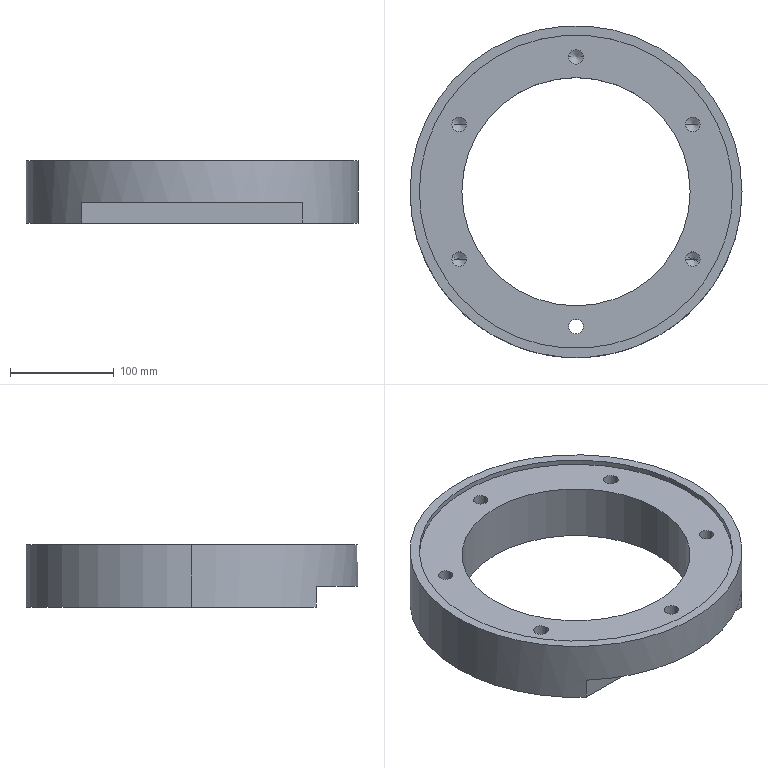Component | SolidWorks | JF21-80.1-1-3(_)-1-SOLID31-1 | 1 solid | 33 faces | box 320 x 320 x 60 mm | volume 2225570 mm3 | cylinder 18 | cone 10 | plane 5 | commonest cylinder face diameters 14 x12 302 x2 320 x2 220 x2
STEP:
#1=COLOUR_RGB('',0.7922,0.8196,0.9333);
#2=FILL_AREA_STYLE_COLOUR('',#1);
#3=FILL_AREA_STYLE('',(#2));
#4=SURFACE_STYLE_FILL_AREA(#3);
#5=SURFACE_SIDE_STYLE('',(#4));
#6=SURFACE_STYLE_USAGE(.BOTH.,#5);
#7=PRESENTATION_STYLE_ASSIGNMENT((#6));
#8=CARTESIAN_POINT('',(-4.708,-13.039,24.961));
#9=VERTEX_POINT('',#8);
#10=CARTESIAN_POINT('',(-4.157,-13.039,24.961));
#11=VERTEX_POINT('',#10);
#12=CARTESIAN_POINT('',(-4.432,-13.039,24.961));
#13=DIRECTION('',(0.,0.,1.));
#14=DIRECTION('',(1.,0.,0.));
#15=AXIS2_PLACEMENT_3D('',#12,#13,#14);
#16=CIRCLE('',#15,0.2756);
#17=EDGE_CURVE('',#9,#11,#16,.T.);
#18=ORIENTED_EDGE('',*,*,#17,.F.);
#19=CARTESIAN_POINT('',(-4.708,-13.039,26.378));
#20=VERTEX_POINT('',#19);
#21=CARTESIAN_POINT('',(-4.708,-13.039,26.378));
#22=DIRECTION('',(0.,0.,1.));
#23=VECTOR('',#22,39.37);
#24=LINE('',#21,#23);
#25=EDGE_CURVE('',#9,#20,#24,.T.);
#26=ORIENTED_EDGE('',*,*,#25,.T.);
#27=CARTESIAN_POINT('',(-4.157,-13.039,26.378));
#28=VERTEX_POINT('',#27);
#29=CARTESIAN_POINT('',(-4.432,-13.039,26.378));
#30=DIRECTION('',(0.,0.,1.));
#31=DIRECTION('',(1.,0.,0.));
#32=AXIS2_PLACEMENT_3D('',#29,#30,#31);
#33=CIRCLE('',#32,0.2756);
#34=EDGE_CURVE('',#20,#28,#33,.T.);
#35=ORIENTED_EDGE('',*,*,#34,.T.);
#36=CARTESIAN_POINT('',(-4.157,-13.039,26.378));
#37=DIRECTION('',(0.,0.,1.));
#38=VECTOR('',#37,39.37);
#39=LINE('',#36,#38);
#40=EDGE_CURVE('',#11,#28,#39,.T.);
#41=ORIENTED_EDGE('',*,*,#40,.F.);
#42=EDGE_LOOP('',(#18,#26,#35,#41));
#43=FACE_OUTER_BOUND('',#42,.T.);
#44=CARTESIAN_POINT('',(-4.432,-13.039,26.378));
#45=DIRECTION('',(0.,0.,1.));
#46=DIRECTION('',(-1.,0.,0.));
#47=AXIS2_PLACEMENT_3D('',#44,#45,#46);
#48=CYLINDRICAL_SURFACE('',#47,0.2756);
#49=ADVANCED_FACE('',(#43),#48,.F.);
#50=CARTESIAN_POINT('',(-4.432,-13.039,24.795));
#51=VERTEX_POINT('',#50);
#52=CARTESIAN_POINT('',(-4.157,-13.039,24.961));
#53=DIRECTION('',(0.8572,0.,0.515));
#54=VECTOR('',#53,39.37);
#55=LINE('',#52,#54);
#56=EDGE_CURVE('',#51,#11,#55,.T.);
#57=ORIENTED_EDGE('',*,*,#56,.F.);
#58=CARTESIAN_POINT('',(-4.708,-13.039,24.961));
#59=DIRECTION('',(-0.8572,0.,0.515));
#60=VECTOR('',#59,39.37);
#61=LINE('',#58,#60);
#62=EDGE_CURVE('',#51,#9,#61,.T.);
#63=ORIENTED_EDGE('',*,*,#62,.T.);
#64=ORIENTED_EDGE('',*,*,#17,.T.);
#65=EDGE_LOOP('',(#57,#63,#64));
#66=FACE_OUTER_BOUND('',#65,.T.);
#67=CARTESIAN_POINT('',(-4.432,-13.039,24.961));
#68=DIRECTION('',(0.,0.,1.));
#69=DIRECTION('',(-1.,0.,0.));
#70=AXIS2_PLACEMENT_3D('',#67,#68,#69);
#71=CONICAL_SURFACE('',#70,0.2756,1.03);
#72=ADVANCED_FACE('',(#66),#71,.F.);
#73=CARTESIAN_POINT('',(-4.708,-18.157,24.961));
#74=VERTEX_POINT('',#73);
#75=CARTESIAN_POINT('',(-4.157,-18.157,24.961));
#76=VERTEX_POINT('',#75);
#77=CARTESIAN_POINT('',(-4.432,-18.157,24.961));
#78=DIRECTION('',(0.,0.,1.));
#79=DIRECTION('',(1.,0.,0.));
#80=AXIS2_PLACEMENT_3D('',#77,#78,#79);
#81=CIRCLE('',#80,0.2756);
#82=EDGE_CURVE('',#74,#76,#81,.T.);
#83=ORIENTED_EDGE('',*,*,#82,.F.);
#84=CARTESIAN_POINT('',(-4.708,-18.157,26.378));
#85=VERTEX_POINT('',#84);
#86=CARTESIAN_POINT('',(-4.708,-18.157,26.378));
#87=DIRECTION('',(0.,0.,1.));
#88=VECTOR('',#87,39.37);
#89=LINE('',#86,#88);
#90=EDGE_CURVE('',#74,#85,#89,.T.);
#91=ORIENTED_EDGE('',*,*,#90,.T.);
#92=CARTESIAN_POINT('',(-4.157,-18.157,26.378));
#93=VERTEX_POINT('',#92);
#94=CARTESIAN_POINT('',(-4.432,-18.157,26.378));
#95=DIRECTION('',(0.,0.,1.));
#96=DIRECTION('',(1.,0.,0.));
#97=AXIS2_PLACEMENT_3D('',#94,#95,#96);
#98=CIRCLE('',#97,0.2756);
#99=EDGE_CURVE('',#85,#93,#98,.T.);
#100=ORIENTED_EDGE('',*,*,#99,.T.);
#101=CARTESIAN_POINT('',(-4.157,-18.157,26.378));
#102=DIRECTION('',(0.,0.,1.));
#103=VECTOR('',#102,39.37);
#104=LINE('',#101,#103);
#105=EDGE_CURVE('',#76,#93,#104,.T.);
#106=ORIENTED_EDGE('',*,*,#105,.F.);
#107=EDGE_LOOP('',(#83,#91,#100,#106));
#108=FACE_OUTER_BOUND('',#107,.T.);
#109=CARTESIAN_POINT('',(-4.432,-18.157,26.378));
#110=DIRECTION('',(0.,0.,1.));
#111=DIRECTION('',(-1.,0.,0.));
#112=AXIS2_PLACEMENT_3D('',#109,#110,#111);
#113=CYLINDRICAL_SURFACE('',#112,0.2756);
#114=ADVANCED_FACE('',(#108),#113,.F.);
#115=CARTESIAN_POINT('',(-4.432,-18.157,24.795));
#116=VERTEX_POINT('',#115);
#117=CARTESIAN_POINT('',(-4.157,-18.157,24.961));
#118=DIRECTION('',(0.8572,0.,0.515));
#119=VECTOR('',#118,39.37);
#120=LINE('',#117,#119);
#121=EDGE_CURVE('',#116,#76,#120,.T.);
#122=ORIENTED_EDGE('',*,*,#121,.F.);
#123=CARTESIAN_POINT('',(-4.708,-18.157,24.961));
#124=DIRECTION('',(-0.8572,0.,0.515));
#125=VECTOR('',#124,39.37);
#126=LINE('',#123,#125);
#127=EDGE_CURVE('',#116,#74,#126,.T.);
#128=ORIENTED_EDGE('',*,*,#127,.T.);
#129=ORIENTED_EDGE('',*,*,#82,.T.);
#130=EDGE_LOOP('',(#122,#128,#129));
#131=FACE_OUTER_BOUND('',#130,.T.);
#132=CARTESIAN_POINT('',(-4.432,-18.157,24.961));
#133=DIRECTION('',(0.,0.,1.));
#134=DIRECTION('',(-1.,0.,0.));
#135=AXIS2_PLACEMENT_3D('',#132,#133,#134);
#136=CONICAL_SURFACE('',#135,0.2756,1.03);
#137=ADVANCED_FACE('',(#131),#136,.F.);
#138=CARTESIAN_POINT('',(4.157,-18.157,24.961));
#139=VERTEX_POINT('',#138);
#140=CARTESIAN_POINT('',(4.708,-18.157,24.961));
#141=VERTEX_POINT('',#140);
#142=CARTESIAN_POINT('',(4.432,-18.157,24.961));
#143=DIRECTION('',(0.,0.,1.));
#144=DIRECTION('',(1.,0.,0.));
#145=AXIS2_PLACEMENT_3D('',#142,#143,#144);
#146=CIRCLE('',#145,0.2756);
#147=EDGE_CURVE('',#139,#141,#146,.T.);
#148=ORIENTED_EDGE('',*,*,#147,.F.);
#149=CARTESIAN_POINT('',(4.157,-18.157,26.378));
#150=VERTEX_POINT('',#149);
#151=CARTESIAN_POINT('',(4.157,-18.157,26.378));
#152=DIRECTION('',(0.,0.,1.));
#153=VECTOR('',#152,39.37);
#154=LINE('',#151,#153);
#155=EDGE_CURVE('',#139,#150,#154,.T.);
#156=ORIENTED_EDGE('',*,*,#155,.T.);
#157=CARTESIAN_POINT('',(4.708,-18.157,26.378));
#158=VERTEX_POINT('',#157);
#159=CARTESIAN_POINT('',(4.432,-18.157,26.378));
#160=DIRECTION('',(0.,0.,1.));
#161=DIRECTION('',(1.,0.,0.));
#162=AXIS2_PLACEMENT_3D('',#159,#160,#161);
#163=CIRCLE('',#162,0.2756);
#164=EDGE_CURVE('',#150,#158,#163,.T.);
#165=ORIENTED_EDGE('',*,*,#164,.T.);
#166=CARTESIAN_POINT('',(4.708,-18.157,26.378));
#167=DIRECTION('',(0.,0.,1.));
#168=VECTOR('',#167,39.37);
#169=LINE('',#166,#168);
#170=EDGE_CURVE('',#141,#158,#169,.T.);
#171=ORIENTED_EDGE('',*,*,#170,.F.);
#172=EDGE_LOOP('',(#148,#156,#165,#171));
#173=FACE_OUTER_BOUND('',#172,.T.);
#174=CARTESIAN_POINT('',(4.432,-18.157,26.378));
#175=DIRECTION('',(0.,0.,1.));
#176=DIRECTION('',(-1.,0.,0.));
#177=AXIS2_PLACEMENT_3D('',#174,#175,#176);
#178=CYLINDRICAL_SURFACE('',#177,0.2756);
#179=ADVANCED_FACE('',(#173),#178,.F.);
#180=CARTESIAN_POINT('',(4.432,-18.157,24.795));
#181=VERTEX_POINT('',#180);
#182=CARTESIAN_POINT('',(4.708,-18.157,24.961));
#183=DIRECTION('',(0.8572,0.,0.515));
#184=VECTOR('',#183,39.37);
#185=LINE('',#182,#184);
#186=EDGE_CURVE('',#181,#141,#185,.T.);
#187=ORIENTED_EDGE('',*,*,#186,.F.);
#188=CARTESIAN_POINT('',(4.157,-18.157,24.961));
#189=DIRECTION('',(-0.8572,0.,0.515));
#190=VECTOR('',#189,39.37);
#191=LINE('',#188,#190);
#192=EDGE_CURVE('',#181,#139,#191,.T.);
#193=ORIENTED_EDGE('',*,*,#192,.T.);
#194=ORIENTED_EDGE('',*,*,#147,.T.);
#195=EDGE_LOOP('',(#187,#193,#194));
#196=FACE_OUTER_BOUND('',#195,.T.);
#197=CARTESIAN_POINT('',(4.432,-18.157,24.961));
#198=DIRECTION('',(0.,0.,1.));
#199=DIRECTION('',(-1.,0.,0.));
#200=AXIS2_PLACEMENT_3D('',#197,#198,#199);
#201=CONICAL_SURFACE('',#200,0.2756,1.03);
#202=ADVANCED_FACE('',(#196),#201,.F.);
#203=CARTESIAN_POINT('',(4.157,-13.039,24.961));
#204=VERTEX_POINT('',#203);
#205=CARTESIAN_POINT('',(4.708,-13.039,24.961));
#206=VERTEX_POINT('',#205);
#207=CARTESIAN_POINT('',(4.432,-13.039,24.961));
#208=DIRECTION('',(0.,0.,1.));
#209=DIRECTION('',(1.,0.,0.));
#210=AXIS2_PLACEMENT_3D('',#207,#208,#209);
#211=CIRCLE('',#210,0.2756);
#212=EDGE_CURVE('',#204,#206,#211,.T.);
#213=ORIENTED_EDGE('',*,*,#212,.F.);
#214=CARTESIAN_POINT('',(4.157,-13.039,26.378));
#215=VERTEX_POINT('',#214);
#216=CARTESIAN_POINT('',(4.157,-13.039,26.378));
#217=DIRECTION('',(0.,0.,1.));
#218=VECTOR('',#217,39.37);
#219=LINE('',#216,#218);
#220=EDGE_CURVE('',#204,#215,#219,.T.);
#221=ORIENTED_EDGE('',*,*,#220,.T.);
#222=CARTESIAN_POINT('',(4.708,-13.039,26.378));
#223=VERTEX_POINT('',#222);
#224=CARTESIAN_POINT('',(4.432,-13.039,26.378));
#225=DIRECTION('',(0.,0.,1.));
#226=DIRECTION('',(1.,0.,0.));
#227=AXIS2_PLACEMENT_3D('',#224,#225,#226);
#228=CIRCLE('',#227,0.2756);
#229=EDGE_CURVE('',#215,#223,#228,.T.);
#230=ORIENTED_EDGE('',*,*,#229,.T.);
#231=CARTESIAN_POINT('',(4.708,-13.039,26.378));
#232=DIRECTION('',(0.,0.,1.));
#233=VECTOR('',#232,39.37);
#234=LINE('',#231,#233);
#235=EDGE_CURVE('',#206,#223,#234,.T.);
#236=ORIENTED_EDGE('',*,*,#235,.F.);
#237=EDGE_LOOP('',(#213,#221,#230,#236));
#238=FACE_OUTER_BOUND('',#237,.T.);
#239=CARTESIAN_POINT('',(4.432,-13.039,26.378));
#240=DIRECTION('',(0.,0.,1.));
#241=DIRECTION('',(-1.,0.,0.));
#242=AXIS2_PLACEMENT_3D('',#239,#240,#241);
#243=CYLINDRICAL_SURFACE('',#242,0.2756);
#244=ADVANCED_FACE('',(#238),#243,.F.);
#245=CARTESIAN_POINT('',(4.432,-13.039,24.795));
#246=VERTEX_POINT('',#245);
#247=CARTESIAN_POINT('',(4.708,-13.039,24.961));
#248=DIRECTION('',(0.8572,0.,0.515));
#249=VECTOR('',#248,39.37);
#250=LINE('',#247,#249);
#251=EDGE_CURVE('',#246,#206,#250,.T.);
#252=ORIENTED_EDGE('',*,*,#251,.F.);
#253=CARTESIAN_POINT('',(4.157,-13.039,24.961));
#254=DIRECTION('',(-0.8572,0.,0.515));
#255=VECTOR('',#254,39.37);
#256=LINE('',#253,#255);
#257=EDGE_CURVE('',#246,#204,#256,.T.);
#258=ORIENTED_EDGE('',*,*,#257,.T.);
#259=ORIENTED_EDGE('',*,*,#212,.T.);
#260=EDGE_LOOP('',(#252,#258,#259));
#261=FACE_OUTER_BOUND('',#260,.T.);
#262=CARTESIAN_POINT('',(4.432,-13.039,24.961));
#263=DIRECTION('',(0.,0.,1.));
#264=DIRECTION('',(-1.,0.,0.));
#265=AXIS2_PLACEMENT_3D('',#262,#263,#264);
#266=CONICAL_SURFACE('',#265,0.2756,1.03);
#267=ADVANCED_FACE('',(#261),#266,.F.);
#268=CARTESIAN_POINT('',(-0.2756,-10.48,24.961));
#269=VERTEX_POINT('',#268);
#270=CARTESIAN_POINT('',(0.2756,-10.48,24.961));
#271=VERTEX_POINT('',#270);
#272=CARTESIAN_POINT('',(0.,-10.48,24.961));
#273=DIRECTION('',(0.,0.,1.));
#274=DIRECTION('',(1.,0.,0.));
#275=AXIS2_PLACEMENT_3D('',#272,#273,#274);
#276=CIRCLE('',#275,0.2756);
#277=EDGE_CURVE('',#269,#271,#276,.T.);
#278=ORIENTED_EDGE('',*,*,#277,.F.);
#279=CARTESIAN_POINT('',(-0.2756,-10.48,26.378));
#280=VERTEX_POINT('',#279);
#281=CARTESIAN_POINT('',(-0.2756,-10.48,26.378));
#282=DIRECTION('',(0.,0.,1.));
#283=VECTOR('',#282,39.37);
#284=LINE('',#281,#283);
#285=EDGE_CURVE('',#269,#280,#284,.T.);
#286=ORIENTED_EDGE('',*,*,#285,.T.);
#287=CARTESIAN_POINT('',(0.2756,-10.48,26.378));
#288=VERTEX_POINT('',#287);
#289=CARTESIAN_POINT('',(0.,-10.48,26.378));
#290=DIRECTION('',(0.,0.,1.));
#291=DIRECTION('',(1.,0.,0.));
#292=AXIS2_PLACEMENT_3D('',#289,#290,#291);
#293=CIRCLE('',#292,0.2756);
#294=EDGE_CURVE('',#280,#288,#293,.T.);
#295=ORIENTED_EDGE('',*,*,#294,.T.);
#296=CARTESIAN_POINT('',(0.2756,-10.48,26.378));
#297=DIRECTION('',(0.,0.,1.));
#298=VECTOR('',#297,39.37);
#299=LINE('',#296,#298);
#300=EDGE_CURVE('',#271,#288,#299,.T.);
#301=ORIENTED_EDGE('',*,*,#300,.F.);
#302=EDGE_LOOP('',(#278,#286,#295,#301));
#303=FACE_OUTER_BOUND('',#302,.T.);
#304=CARTESIAN_POINT('',(0.,-10.48,26.378));
#305=DIRECTION('',(0.,0.,1.));
#306=DIRECTION('',(-1.,0.,0.));
#307=AXIS2_PLACEMENT_3D('',#304,#305,#306);
#308=CYLINDRICAL_SURFACE('',#307,0.2756);
#309=ADVANCED_FACE('',(#303),#308,.F.);
#310=CARTESIAN_POINT('',(-0.,-10.48,24.795));
#311=VERTEX_POINT('',#310);
#312=CARTESIAN_POINT('',(0.2756,-10.48,24.961));
#313=DIRECTION('',(0.8572,0.,0.515));
#314=VECTOR('',#313,39.37);
#315=LINE('',#312,#314);
#316=EDGE_CURVE('',#311,#271,#315,.T.);
#317=ORIENTED_EDGE('',*,*,#316,.F.);
#318=CARTESIAN_POINT('',(-0.2756,-10.48,24.961));
#319=DIRECTION('',(-0.8572,0.,0.515));
#320=VECTOR('',#319,39.37);
#321=LINE('',#318,#320);
#322=EDGE_CURVE('',#311,#269,#321,.T.);
#323=ORIENTED_EDGE('',*,*,#322,.T.);
#324=ORIENTED_EDGE('',*,*,#277,.T.);
#325=EDGE_LOOP('',(#317,#323,#324));
#326=FACE_OUTER_BOUND('',#325,.T.);
#327=CARTESIAN_POINT('',(0.,-10.48,24.961));
#328=DIRECTION('',(0.,0.,1.));
#329=DIRECTION('',(-1.,0.,0.));
#330=AXIS2_PLACEMENT_3D('',#327,#328,#329);
#331=CONICAL_SURFACE('',#330,0.2756,1.03);
#332=ADVANCED_FACE('',(#326),#331,.F.);
#333=CARTESIAN_POINT('',(-5.945,-15.598,26.378));
#334=VERTEX_POINT('',#333);
#335=CARTESIAN_POINT('',(5.945,-15.598,26.378));
#336=VERTEX_POINT('',#335);
#337=CARTESIAN_POINT('',(0.,-15.598,26.378));
#338=DIRECTION('',(0.,0.,1.));
#339=DIRECTION('',(1.,0.,0.));
#340=AXIS2_PLACEMENT_3D('',#337,#338,#339);
#341=CIRCLE('',#340,5.945);
#342=EDGE_CURVE('',#334,#336,#341,.T.);
#343=ORIENTED_EDGE('',*,*,#342,.F.);
#344=CARTESIAN_POINT('',(-5.945,-15.598,26.575));
#345=VERTEX_POINT('',#344);
#346=CARTESIAN_POINT('',(-5.945,-15.598,26.378));
#347=DIRECTION('',(0.,0.,1.));
#348=VECTOR('',#347,39.37);
#349=LINE('',#346,#348);
#350=EDGE_CURVE('',#334,#345,#349,.T.);
#351=ORIENTED_EDGE('',*,*,#350,.T.);
#352=CARTESIAN_POINT('',(5.945,-15.598,26.575));
#353=VERTEX_POINT('',#352);
#354=CARTESIAN_POINT('',(0.,-15.598,26.575));
#355=DIRECTION('',(0.,0.,1.));
#356=DIRECTION('',(1.,0.,0.));
#357=AXIS2_PLACEMENT_3D('',#354,#355,#356);
#358=CIRCLE('',#357,5.945);
#359=EDGE_CURVE('',#345,#353,#358,.T.);
#360=ORIENTED_EDGE('',*,*,#359,.T.);
#361=CARTESIAN_POINT('',(5.945,-15.598,26.378));
#362=DIRECTION('',(0.,0.,1.));
#363=VECTOR('',#362,39.37);
#364=LINE('',#361,#363);
#365=EDGE_CURVE('',#336,#353,#364,.T.);
#366=ORIENTED_EDGE('',*,*,#365,.F.);
#367=EDGE_LOOP('',(#343,#351,#360,#366));
#368=FACE_OUTER_BOUND('',#367,.T.);
#369=CARTESIAN_POINT('',(0.,-15.598,26.378));
#370=DIRECTION('',(0.,0.,1.));
#371=DIRECTION('',(-1.,0.,0.));
#372=AXIS2_PLACEMENT_3D('',#369,#370,#371);
#373=CYLINDRICAL_SURFACE('',#372,5.945);
#374=ADVANCED_FACE('',(#368),#373,.F.);
#375=CARTESIAN_POINT('',(6.299,-15.598,24.213));
#376=VERTEX_POINT('',#375);
#377=CARTESIAN_POINT('',(-6.299,-15.598,24.213));
#378=VERTEX_POINT('',#377);
#379=CARTESIAN_POINT('',(0.,-15.598,24.213));
#380=DIRECTION('',(0.,0.,1.));
#381=DIRECTION('',(1.,0.,0.));
#382=AXIS2_PLACEMENT_3D('',#379,#380,#381);
#383=CIRCLE('',#382,6.299);
#384=EDGE_CURVE('',#376,#378,#383,.T.);
#385=ORIENTED_EDGE('',*,*,#384,.T.);
#386=CARTESIAN_POINT('',(-6.299,-15.598,26.575));
#387=VERTEX_POINT('',#386);
#388=CARTESIAN_POINT('',(-6.299,-15.598,24.213));
#389=DIRECTION('',(0.,0.,1.));
#390=VECTOR('',#389,39.37);
#391=LINE('',#388,#390);
#392=EDGE_CURVE('',#378,#387,#391,.T.);
#393=ORIENTED_EDGE('',*,*,#392,.T.);
#394=CARTESIAN_POINT('',(6.299,-15.598,26.575));
#395=VERTEX_POINT('',#394);
#396=CARTESIAN_POINT('',(0.,-15.598,26.575));
#397=DIRECTION('',(0.,0.,1.));
#398=DIRECTION('',(1.,0.,0.));
#399=AXIS2_PLACEMENT_3D('',#396,#397,#398);
#400=CIRCLE('',#399,6.299);
#401=EDGE_CURVE('',#395,#387,#400,.T.);
#402=ORIENTED_EDGE('',*,*,#401,.F.);
#403=CARTESIAN_POINT('',(6.299,-15.598,24.213));
#404=DIRECTION('',(0.,0.,1.));
#405=VECTOR('',#404,39.37);
#406=LINE('',#403,#405);
#407=EDGE_CURVE('',#376,#395,#406,.T.);
#408=ORIENTED_EDGE('',*,*,#407,.F.);
#409=EDGE_LOOP('',(#385,#393,#402,#408));
#410=FACE_OUTER_BOUND('',#409,.T.);
#411=CARTESIAN_POINT('',(0.,-15.598,24.213));
#412=DIRECTION('',(0.,0.,1.));
#413=DIRECTION('',(-1.,0.,0.));
#414=AXIS2_PLACEMENT_3D('',#411,#412,#413);
#415=CYLINDRICAL_SURFACE('',#414,6.299);
#416=ADVANCED_FACE('',(#410),#415,.T.);
#417=CARTESIAN_POINT('',(-4.331,-15.598,24.213));
#418=VERTEX_POINT('',#417);
#419=CARTESIAN_POINT('',(4.331,-15.598,24.213));
#420=VERTEX_POINT('',#419);
#421=CARTESIAN_POINT('',(0.,-15.598,24.213));
#422=DIRECTION('',(0.,0.,1.));
#423=DIRECTION('',(1.,0.,0.));
#424=AXIS2_PLACEMENT_3D('',#421,#422,#423);
#425=CIRCLE('',#424,4.331);
#426=EDGE_CURVE('',#418,#420,#425,.T.);
#427=ORIENTED_EDGE('',*,*,#426,.F.);
#428=CARTESIAN_POINT('',(-4.331,-15.598,26.378));
#429=VERTEX_POINT('',#428);
#430=CARTESIAN_POINT('',(-4.331,-15.598,24.213));
#431=DIRECTION('',(0.,0.,1.));
#432=VECTOR('',#431,39.37);
#433=LINE('',#430,#432);
#434=EDGE_CURVE('',#418,#429,#433,.T.);
#435=ORIENTED_EDGE('',*,*,#434,.T.);
#436=CARTESIAN_POINT('',(4.331,-15.598,26.378));
#437=VERTEX_POINT('',#436);
#438=CARTESIAN_POINT('',(0.,-15.598,26.378));
#439=DIRECTION('',(0.,0.,-1.));
#440=DIRECTION('',(1.,0.,0.));
#441=AXIS2_PLACEMENT_3D('',#438,#439,#440);
#442=CIRCLE('',#441,4.331);
#443=EDGE_CURVE('',#437,#429,#442,.T.);
#444=ORIENTED_EDGE('',*,*,#443,.F.);
#445=CARTESIAN_POINT('',(4.331,-15.598,24.213));
#446=DIRECTION('',(0.,0.,1.));
#447=VECTOR('',#446,39.37);
#448=LINE('',#445,#447);
#449=EDGE_CURVE('',#420,#437,#448,.T.);
#450=ORIENTED_EDGE('',*,*,#449,.F.);
#451=EDGE_LOOP('',(#427,#435,#444,#450));
#452=FACE_OUTER_BOUND('',#451,.T.);
#453=CARTESIAN_POINT('',(0.,-15.598,24.213));
#454=DIRECTION('',(0.,0.,1.));
#455=DIRECTION('',(-1.,0.,0.));
#456=AXIS2_PLACEMENT_3D('',#453,#454,#455);
#457=CYLINDRICAL_SURFACE('',#456,4.331);
#458=ADVANCED_FACE('',(#452),#457,.F.);
#459=CARTESIAN_POINT('',(-0.2756,-20.716,25.));
#460=VERTEX_POINT('',#459);
#461=CARTESIAN_POINT('',(0.2756,-20.716,25.));
#462=VERTEX_POINT('',#461);
#463=CARTESIAN_POINT('',(-0.,-20.716,25.));
#464=DIRECTION('',(0.,0.,1.));
#465=DIRECTION('',(-1.,0.,0.));
#466=AXIS2_PLACEMENT_3D('',#463,#464,#465);
#467=CIRCLE('',#466,0.2756);
#468=EDGE_CURVE('',#460,#462,#467,.T.);
#469=ORIENTED_EDGE('',*,*,#468,.F.);
#470=CARTESIAN_POINT('',(-0.2756,-20.716,26.378));
#471=VERTEX_POINT('',#470);
#472=CARTESIAN_POINT('',(-0.2756,-20.716,26.378));
#473=DIRECTION('',(0.,0.,1.));
#474=VECTOR('',#473,39.37);
#475=LINE('',#472,#474);
#476=EDGE_CURVE('',#460,#471,#475,.T.);
#477=ORIENTED_EDGE('',*,*,#476,.T.);
#478=CARTESIAN_POINT('',(0.2756,-20.716,26.378));
#479=VERTEX_POINT('',#478);
#480=CARTESIAN_POINT('',(-0.,-20.716,26.378));
#481=DIRECTION('',(0.,0.,1.));
#482=DIRECTION('',(1.,0.,0.));
#483=AXIS2_PLACEMENT_3D('',#480,#481,#482);
#484=CIRCLE('',#483,0.2756);
#485=EDGE_CURVE('',#471,#479,#484,.T.);
#486=ORIENTED_EDGE('',*,*,#485,.T.);
#487=CARTESIAN_POINT('',(0.2756,-20.716,26.378));
#488=DIRECTION('',(0.,0.,1.));
#489=VECTOR('',#488,39.37);
#490=LINE('',#487,#489);
#491=EDGE_CURVE('',#462,#479,#490,.T.);
#492=ORIENTED_EDGE('',*,*,#491,.F.);
#493=EDGE_LOOP('',(#469,#477,#486,#492));
#494=FACE_OUTER_BOUND('',#493,.T.);
#495=CARTESIAN_POINT('',(-0.,-20.716,26.378));
#496=DIRECTION('',(0.,0.,1.));
#497=DIRECTION('',(-1.,0.,0.));
#498=AXIS2_PLACEMENT_3D('',#495,#496,#497);
#499=CYLINDRICAL_SURFACE('',#498,0.2756);
#500=ADVANCED_FACE('',(#494),#499,.F.);
#501=ORIENTED_EDGE('',*,*,#476,.F.);
#502=CARTESIAN_POINT('',(-0.,-20.716,25.));
#503=DIRECTION('',(0.,0.,1.));
#504=DIRECTION('',(-1.,0.,0.));
#505=AXIS2_PLACEMENT_3D('',#502,#503,#504);
#506=CIRCLE('',#505,0.2756);
#507=EDGE_CURVE('',#462,#460,#506,.T.);
#508=ORIENTED_EDGE('',*,*,#507,.F.);
#509=ORIENTED_EDGE('',*,*,#491,.T.);
#510=CARTESIAN_POINT('',(-0.,-20.716,26.378));
#511=DIRECTION('',(0.,0.,1.));
#512=DIRECTION('',(1.,0.,0.));
#513=AXIS2_PLACEMENT_3D('',#510,#511,#512);
#514=CIRCLE('',#513,0.2756);
#515=EDGE_CURVE('',#479,#471,#514,.T.);
#516=ORIENTED_EDGE('',*,*,#515,.T.);
#517=EDGE_LOOP('',(#501,#508,#509,#516));
#518=FACE_OUTER_BOUND('',#517,.T.);
#519=CARTESIAN_POINT('',(-0.,-20.716,26.378));
#520=DIRECTION('',(0.,0.,1.));
#521=DIRECTION('',(-1.,0.,0.));
#522=AXIS2_PLACEMENT_3D('',#519,#520,#521);
#523=CYLINDRICAL_SURFACE('',#522,0.2756);
#524=ADVANCED_FACE('',(#518),#523,.F.);
#525=ORIENTED_EDGE('',*,*,#434,.F.);
#526=CARTESIAN_POINT('',(0.,-15.598,24.213));
#527=DIRECTION('',(0.,0.,1.));
#528=DIRECTION('',(1.,0.,0.));
#529=AXIS2_PLACEMENT_3D('',#526,#527,#528);
#530=CIRCLE('',#529,4.331);
#531=EDGE_CURVE('',#420,#418,#530,.T.);
#532=ORIENTED_EDGE('',*,*,#531,.F.);
#533=ORIENTED_EDGE('',*,*,#449,.T.);
#534=CARTESIAN_POINT('',(0.,-15.598,26.378));
#535=DIRECTION('',(0.,0.,-1.));
#536=DIRECTION('',(1.,0.,0.));
#537=AXIS2_PLACEMENT_3D('',#534,#535,#536);
#538=CIRCLE('',#537,4.331);
#539=EDGE_CURVE('',#429,#437,#538,.T.);
#540=ORIENTED_EDGE('',*,*,#539,.F.);
#541=EDGE_LOOP('',(#525,#532,#533,#540));
#542=FACE_OUTER_BOUND('',#541,.T.);
#543=CARTESIAN_POINT('',(0.,-15.598,24.213));
#544=DIRECTION('',(0.,0.,1.));
#545=DIRECTION('',(-1.,0.,0.));
#546=AXIS2_PLACEMENT_3D('',#543,#544,#545);
#547=CYLINDRICAL_SURFACE('',#546,4.331);
#548=ADVANCED_FACE('',(#542),#547,.F.);
#549=ORIENTED_EDGE('',*,*,#392,.F.);
#550=CARTESIAN_POINT('',(-4.175,-20.315,24.213));
#551=VERTEX_POINT('',#550);
#552=CARTESIAN_POINT('',(0.,-15.598,24.213));
#553=DIRECTION('',(0.,0.,1.));
#554=DIRECTION('',(1.,0.,0.));
#555=AXIS2_PLACEMENT_3D('',#552,#553,#554);
#556=CIRCLE('',#555,6.299);
#557=EDGE_CURVE('',#378,#551,#556,.T.);
#558=ORIENTED_EDGE('',*,*,#557,.T.);
#559=CARTESIAN_POINT('',(-4.175,-20.315,25.));
#560=VERTEX_POINT('',#559);
#561=CARTESIAN_POINT('',(-4.175,-20.315,25.));
#562=DIRECTION('',(0.,0.,1.));
#563=VECTOR('',#562,39.37);
#564=LINE('',#561,#563);
#565=EDGE_CURVE('',#551,#560,#564,.T.);
#566=ORIENTED_EDGE('',*,*,#565,.T.);
#567=CARTESIAN_POINT('',(4.175,-20.315,25.));
#568=VERTEX_POINT('',#567);
#569=CARTESIAN_POINT('',(0.,-15.598,25.));
#570=DIRECTION('',(0.,0.,-1.));
#571=DIRECTION('',(-1.,0.,0.));
#572=AXIS2_PLACEMENT_3D('',#569,#570,#571);
#573=CIRCLE('',#572,6.299);
#574=EDGE_CURVE('',#568,#560,#573,.T.);
#575=ORIENTED_EDGE('',*,*,#574,.F.);
#576=CARTESIAN_POINT('',(4.175,-20.315,24.213));
#577=VERTEX_POINT('',#576);
#578=CARTESIAN_POINT('',(4.175,-20.315,25.));
#579=DIRECTION('',(0.,0.,1.));
#580=VECTOR('',#579,39.37);
#581=LINE('',#578,#580);
#582=EDGE_CURVE('',#577,#568,#581,.T.);
#583=ORIENTED_EDGE('',*,*,#582,.F.);
#584=CARTESIAN_POINT('',(0.,-15.598,24.213));
#585=DIRECTION('',(0.,0.,1.));
#586=DIRECTION('',(1.,0.,0.));
#587=AXIS2_PLACEMENT_3D('',#584,#585,#586);
#588=CIRCLE('',#587,6.299);
#589=EDGE_CURVE('',#577,#376,#588,.T.);
#590=ORIENTED_EDGE('',*,*,#589,.T.);
#591=ORIENTED_EDGE('',*,*,#407,.T.);
#592=CARTESIAN_POINT('',(0.,-15.598,26.575));
#593=DIRECTION('',(0.,0.,1.));
#594=DIRECTION('',(1.,0.,0.));
#595=AXIS2_PLACEMENT_3D('',#592,#593,#594);
#596=CIRCLE('',#595,6.299);
#597=EDGE_CURVE('',#387,#395,#596,.T.);
#598=ORIENTED_EDGE('',*,*,#597,.F.);
#599=EDGE_LOOP('',(#549,#558,#566,#575,#583,#590,#591,#598));
#600=FACE_OUTER_BOUND('',#599,.T.);
#601=CARTESIAN_POINT('',(0.,-15.598,24.213));
#602=DIRECTION('',(0.,0.,1.));
#603=DIRECTION('',(-1.,0.,0.));
#604=AXIS2_PLACEMENT_3D('',#601,#602,#603);
#605=CYLINDRICAL_SURFACE('',#604,6.299);
#606=ADVANCED_FACE('',(#600),#605,.T.);
#607=ORIENTED_EDGE('',*,*,#531,.T.);
#608=ORIENTED_EDGE('',*,*,#426,.T.);
#609=EDGE_LOOP('',(#607,#608));
#610=FACE_BOUND('',#609,.T.);
#611=ORIENTED_EDGE('',*,*,#589,.F.);
#612=CARTESIAN_POINT('',(4.175,-20.315,24.213));
#613=DIRECTION('',(1.,0.,0.));
#614=VECTOR('',#613,39.37);
#615=LINE('',#612,#614);
#616=EDGE_CURVE('',#551,#577,#615,.T.);
#617=ORIENTED_EDGE('',*,*,#616,.F.);
#618=ORIENTED_EDGE('',*,*,#557,.F.);
#619=ORIENTED_EDGE('',*,*,#384,.F.);
#620=EDGE_LOOP('',(#611,#617,#618,#619));
#621=FACE_OUTER_BOUND('',#620,.T.);
#622=CARTESIAN_POINT('',(0.,-15.598,24.213));
#623=DIRECTION('',(0.,0.,1.));
#624=DIRECTION('',(-1.,0.,0.));
#625=AXIS2_PLACEMENT_3D('',#622,#623,#624);
#626=PLANE('',#625);
#627=ADVANCED_FACE('',(#610,#621),#626,.F.);
#628=CARTESIAN_POINT('',(0.,-15.598,26.575));
#629=DIRECTION('',(0.,0.,1.));
#630=DIRECTION('',(1.,0.,0.));
#631=AXIS2_PLACEMENT_3D('',#628,#629,#630);
#632=CIRCLE('',#631,5.945);
#633=EDGE_CURVE('',#353,#345,#632,.T.);
#634=ORIENTED_EDGE('',*,*,#633,.F.);
#635=ORIENTED_EDGE('',*,*,#359,.F.);
#636=EDGE_LOOP('',(#634,#635));
#637=FACE_BOUND('',#636,.T.);
#638=ORIENTED_EDGE('',*,*,#401,.T.);
#639=ORIENTED_EDGE('',*,*,#597,.T.);
#640=EDGE_LOOP('',(#638,#639));
#641=FACE_OUTER_BOUND('',#640,.T.);
#642=CARTESIAN_POINT('',(0.,-15.598,26.575));
#643=DIRECTION('',(0.,0.,1.));
#644=DIRECTION('',(-1.,0.,0.));
#645=AXIS2_PLACEMENT_3D('',#642,#643,#644);
#646=PLANE('',#645);
#647=ADVANCED_FACE('',(#637,#641),#646,.T.);
#648=CARTESIAN_POINT('',(-4.432,-13.039,26.378));
#649=DIRECTION('',(0.,0.,1.));
#650=DIRECTION('',(1.,0.,0.));
#651=AXIS2_PLACEMENT_3D('',#648,#649,#650);
#652=CIRCLE('',#651,0.2756);
#653=EDGE_CURVE('',#28,#20,#652,.T.);
#654=ORIENTED_EDGE('',*,*,#653,.F.);
#655=ORIENTED_EDGE('',*,*,#34,.F.);
#656=EDGE_LOOP('',(#654,#655));
#657=FACE_BOUND('',#656,.T.);
#658=CARTESIAN_POINT('',(-4.432,-18.157,26.378));
#659=DIRECTION('',(0.,0.,1.));
#660=DIRECTION('',(1.,0.,0.));
#661=AXIS2_PLACEMENT_3D('',#658,#659,#660);
#662=CIRCLE('',#661,0.2756);
#663=EDGE_CURVE('',#93,#85,#662,.T.);
#664=ORIENTED_EDGE('',*,*,#663,.F.);
#665=ORIENTED_EDGE('',*,*,#99,.F.);
#666=EDGE_LOOP('',(#664,#665));
#667=FACE_BOUND('',#666,.T.);
#668=ORIENTED_EDGE('',*,*,#515,.F.);
#669=ORIENTED_EDGE('',*,*,#485,.F.);
#670=EDGE_LOOP('',(#668,#669));
#671=FACE_BOUND('',#670,.T.);
#672=CARTESIAN_POINT('',(4.432,-18.157,26.378));
#673=DIRECTION('',(0.,0.,1.));
#674=DIRECTION('',(1.,0.,0.));
#675=AXIS2_PLACEMENT_3D('',#672,#673,#674);
#676=CIRCLE('',#675,0.2756);
#677=EDGE_CURVE('',#158,#150,#676,.T.);
#678=ORIENTED_EDGE('',*,*,#677,.F.);
#679=ORIENTED_EDGE('',*,*,#164,.F.);
#680=EDGE_LOOP('',(#678,#679));
#681=FACE_BOUND('',#680,.T.);
#682=CARTESIAN_POINT('',(4.432,-13.039,26.378));
#683=DIRECTION('',(0.,0.,1.));
#684=DIRECTION('',(1.,0.,0.));
#685=AXIS2_PLACEMENT_3D('',#682,#683,#684);
#686=CIRCLE('',#685,0.2756);
#687=EDGE_CURVE('',#223,#215,#686,.T.);
#688=ORIENTED_EDGE('',*,*,#687,.F.);
#689=ORIENTED_EDGE('',*,*,#229,.F.);
#690=EDGE_LOOP('',(#688,#689));
#691=FACE_BOUND('',#690,.T.);
#692=CARTESIAN_POINT('',(0.,-10.48,26.378));
#693=DIRECTION('',(0.,0.,1.));
#694=DIRECTION('',(1.,0.,0.));
#695=AXIS2_PLACEMENT_3D('',#692,#693,#694);
#696=CIRCLE('',#695,0.2756);
#697=EDGE_CURVE('',#288,#280,#696,.T.);
#698=ORIENTED_EDGE('',*,*,#697,.F.);
#699=ORIENTED_EDGE('',*,*,#294,.F.);
#700=EDGE_LOOP('',(#698,#699));
#701=FACE_BOUND('',#700,.T.);
#702=CARTESIAN_POINT('',(0.,-15.598,26.378));
#703=DIRECTION('',(0.,0.,1.));
#704=DIRECTION('',(1.,0.,0.));
#705=AXIS2_PLACEMENT_3D('',#702,#703,#704);
#706=CIRCLE('',#705,5.945);
#707=EDGE_CURVE('',#336,#334,#706,.T.);
#708=ORIENTED_EDGE('',*,*,#707,.T.);
#709=ORIENTED_EDGE('',*,*,#342,.T.);
#710=EDGE_LOOP('',(#708,#709));
#711=FACE_OUTER_BOUND('',#710,.T.);
#712=ORIENTED_EDGE('',*,*,#443,.T.);
#713=ORIENTED_EDGE('',*,*,#539,.T.);
#714=EDGE_LOOP('',(#712,#713));
#715=FACE_BOUND('',#714,.T.);
#716=CARTESIAN_POINT('',(0.,-15.598,26.378));
#717=DIRECTION('',(0.,0.,1.));
#718=DIRECTION('',(-1.,0.,0.));
#719=AXIS2_PLACEMENT_3D('',#716,#717,#718);
#720=PLANE('',#719);
#721=ADVANCED_FACE('',(#657,#667,#671,#681,#691,#701,#711,#715),#720,.T.);
#722=ORIENTED_EDGE('',*,*,#350,.F.);
#723=ORIENTED_EDGE('',*,*,#707,.F.);
#724=ORIENTED_EDGE('',*,*,#365,.T.);
#725=ORIENTED_EDGE('',*,*,#633,.T.);
#726=EDGE_LOOP('',(#722,#723,#724,#725));
#727=FACE_OUTER_BOUND('',#726,.T.);
#728=CARTESIAN_POINT('',(0.,-15.598,26.378));
#729=DIRECTION('',(0.,0.,1.));
#730=DIRECTION('',(-1.,0.,0.));
#731=AXIS2_PLACEMENT_3D('',#728,#729,#730);
#732=CYLINDRICAL_SURFACE('',#731,5.945);
#733=ADVANCED_FACE('',(#727),#732,.F.);
#734=ORIENTED_EDGE('',*,*,#322,.F.);
#735=ORIENTED_EDGE('',*,*,#316,.T.);
#736=CARTESIAN_POINT('',(0.,-10.48,24.961));
#737=DIRECTION('',(0.,0.,1.));
#738=DIRECTION('',(1.,0.,0.));
#739=AXIS2_PLACEMENT_3D('',#736,#737,#738);
#740=CIRCLE('',#739,0.2756);
#741=EDGE_CURVE('',#271,#269,#740,.T.);
#742=ORIENTED_EDGE('',*,*,#741,.T.);
#743=EDGE_LOOP('',(#734,#735,#742));
#744=FACE_OUTER_BOUND('',#743,.T.);
#745=CARTESIAN_POINT('',(0.,-10.48,24.961));
#746=DIRECTION('',(0.,0.,1.));
#747=DIRECTION('',(-1.,0.,0.));
#748=AXIS2_PLACEMENT_3D('',#745,#746,#747);
#749=CONICAL_SURFACE('',#748,0.2756,1.03);
#750=ADVANCED_FACE('',(#744),#749,.F.);
#751=ORIENTED_EDGE('',*,*,#285,.F.);
#752=ORIENTED_EDGE('',*,*,#741,.F.);
#753=ORIENTED_EDGE('',*,*,#300,.T.);
#754=ORIENTED_EDGE('',*,*,#697,.T.);
#755=EDGE_LOOP('',(#751,#752,#753,#754));
#756=FACE_OUTER_BOUND('',#755,.T.);
#757=CARTESIAN_POINT('',(0.,-10.48,26.378));
#758=DIRECTION('',(0.,0.,1.));
#759=DIRECTION('',(-1.,0.,0.));
#760=AXIS2_PLACEMENT_3D('',#757,#758,#759);
#761=CYLINDRICAL_SURFACE('',#760,0.2756);
#762=ADVANCED_FACE('',(#756),#761,.F.);
#763=ORIENTED_EDGE('',*,*,#257,.F.);
#764=ORIENTED_EDGE('',*,*,#251,.T.);
#765=CARTESIAN_POINT('',(4.432,-13.039,24.961));
#766=DIRECTION('',(0.,0.,1.));
#767=DIRECTION('',(1.,0.,0.));
#768=AXIS2_PLACEMENT_3D('',#765,#766,#767);
#769=CIRCLE('',#768,0.2756);
#770=EDGE_CURVE('',#206,#204,#769,.T.);
#771=ORIENTED_EDGE('',*,*,#770,.T.);
#772=EDGE_LOOP('',(#763,#764,#771));
#773=FACE_OUTER_BOUND('',#772,.T.);
#774=CARTESIAN_POINT('',(4.432,-13.039,24.961));
#775=DIRECTION('',(0.,0.,1.));
#776=DIRECTION('',(-1.,0.,0.));
#777=AXIS2_PLACEMENT_3D('',#774,#775,#776);
#778=CONICAL_SURFACE('',#777,0.2756,1.03);
#779=ADVANCED_FACE('',(#773),#778,.F.);
#780=ORIENTED_EDGE('',*,*,#220,.F.);
#781=ORIENTED_EDGE('',*,*,#770,.F.);
#782=ORIENTED_EDGE('',*,*,#235,.T.);
#783=ORIENTED_EDGE('',*,*,#687,.T.);
#784=EDGE_LOOP('',(#780,#781,#782,#783));
#785=FACE_OUTER_BOUND('',#784,.T.);
#786=CARTESIAN_POINT('',(4.432,-13.039,26.378));
#787=DIRECTION('',(0.,0.,1.));
#788=DIRECTION('',(-1.,0.,0.));
#789=AXIS2_PLACEMENT_3D('',#786,#787,#788);
#790=CYLINDRICAL_SURFACE('',#789,0.2756);
#791=ADVANCED_FACE('',(#785),#790,.F.);
#792=ORIENTED_EDGE('',*,*,#192,.F.);
#793=ORIENTED_EDGE('',*,*,#186,.T.);
#794=CARTESIAN_POINT('',(4.432,-18.157,24.961));
#795=DIRECTION('',(0.,0.,1.));
#796=DIRECTION('',(1.,0.,0.));
#797=AXIS2_PLACEMENT_3D('',#794,#795,#796);
#798=CIRCLE('',#797,0.2756);
#799=EDGE_CURVE('',#141,#139,#798,.T.);
#800=ORIENTED_EDGE('',*,*,#799,.T.);
#801=EDGE_LOOP('',(#792,#793,#800));
#802=FACE_OUTER_BOUND('',#801,.T.);
#803=CARTESIAN_POINT('',(4.432,-18.157,24.961));
#804=DIRECTION('',(0.,0.,1.));
#805=DIRECTION('',(-1.,0.,0.));
#806=AXIS2_PLACEMENT_3D('',#803,#804,#805);
#807=CONICAL_SURFACE('',#806,0.2756,1.03);
#808=ADVANCED_FACE('',(#802),#807,.F.);
#809=ORIENTED_EDGE('',*,*,#155,.F.);
#810=ORIENTED_EDGE('',*,*,#799,.F.);
#811=ORIENTED_EDGE('',*,*,#170,.T.);
#812=ORIENTED_EDGE('',*,*,#677,.T.);
#813=EDGE_LOOP('',(#809,#810,#811,#812));
#814=FACE_OUTER_BOUND('',#813,.T.);
#815=CARTESIAN_POINT('',(4.432,-18.157,26.378));
#816=DIRECTION('',(0.,0.,1.));
#817=DIRECTION('',(-1.,0.,0.));
#818=AXIS2_PLACEMENT_3D('',#815,#816,#817);
#819=CYLINDRICAL_SURFACE('',#818,0.2756);
#820=ADVANCED_FACE('',(#814),#819,.F.);
#821=ORIENTED_EDGE('',*,*,#127,.F.);
#822=ORIENTED_EDGE('',*,*,#121,.T.);
#823=CARTESIAN_POINT('',(-4.432,-18.157,24.961));
#824=DIRECTION('',(0.,0.,1.));
#825=DIRECTION('',(1.,0.,0.));
#826=AXIS2_PLACEMENT_3D('',#823,#824,#825);
#827=CIRCLE('',#826,0.2756);
#828=EDGE_CURVE('',#76,#74,#827,.T.);
#829=ORIENTED_EDGE('',*,*,#828,.T.);
#830=EDGE_LOOP('',(#821,#822,#829));
#831=FACE_OUTER_BOUND('',#830,.T.);
#832=CARTESIAN_POINT('',(-4.432,-18.157,24.961));
#833=DIRECTION('',(0.,0.,1.));
#834=DIRECTION('',(-1.,0.,0.));
#835=AXIS2_PLACEMENT_3D('',#832,#833,#834);
#836=CONICAL_SURFACE('',#835,0.2756,1.03);
#837=ADVANCED_FACE('',(#831),#836,.F.);
#838=ORIENTED_EDGE('',*,*,#90,.F.);
#839=ORIENTED_EDGE('',*,*,#828,.F.);
#840=ORIENTED_EDGE('',*,*,#105,.T.);
#841=ORIENTED_EDGE('',*,*,#663,.T.);
#842=EDGE_LOOP('',(#838,#839,#840,#841));
#843=FACE_OUTER_BOUND('',#842,.T.);
#844=CARTESIAN_POINT('',(-4.432,-18.157,26.378));
#845=DIRECTION('',(0.,0.,1.));
#846=DIRECTION('',(-1.,0.,0.));
#847=AXIS2_PLACEMENT_3D('',#844,#845,#846);
#848=CYLINDRICAL_SURFACE('',#847,0.2756);
#849=ADVANCED_FACE('',(#843),#848,.F.);
#850=ORIENTED_EDGE('',*,*,#62,.F.);
#851=ORIENTED_EDGE('',*,*,#56,.T.);
#852=CARTESIAN_POINT('',(-4.432,-13.039,24.961));
#853=DIRECTION('',(0.,0.,1.));
#854=DIRECTION('',(1.,0.,0.));
#855=AXIS2_PLACEMENT_3D('',#852,#853,#854);
#856=CIRCLE('',#855,0.2756);
#857=EDGE_CURVE('',#11,#9,#856,.T.);
#858=ORIENTED_EDGE('',*,*,#857,.T.);
#859=EDGE_LOOP('',(#850,#851,#858));
#860=FACE_OUTER_BOUND('',#859,.T.);
#861=CARTESIAN_POINT('',(-4.432,-13.039,24.961));
#862=DIRECTION('',(0.,0.,1.));
#863=DIRECTION('',(-1.,0.,0.));
#864=AXIS2_PLACEMENT_3D('',#861,#862,#863);
#865=CONICAL_SURFACE('',#864,0.2756,1.03);
#866=ADVANCED_FACE('',(#860),#865,.F.);
#867=ORIENTED_EDGE('',*,*,#25,.F.);
#868=ORIENTED_EDGE('',*,*,#857,.F.);
#869=ORIENTED_EDGE('',*,*,#40,.T.);
#870=ORIENTED_EDGE('',*,*,#653,.T.);
#871=EDGE_LOOP('',(#867,#868,#869,#870));
#872=FACE_OUTER_BOUND('',#871,.T.);
#873=CARTESIAN_POINT('',(-4.432,-13.039,26.378));
#874=DIRECTION('',(0.,0.,1.));
#875=DIRECTION('',(-1.,0.,0.));
#876=AXIS2_PLACEMENT_3D('',#873,#874,#875);
#877=CYLINDRICAL_SURFACE('',#876,0.2756);
#878=ADVANCED_FACE('',(#872),#877,.F.);
#879=ORIENTED_EDGE('',*,*,#574,.T.);
#880=CARTESIAN_POINT('',(4.175,-20.315,25.));
#881=DIRECTION('',(1.,0.,0.));
#882=VECTOR('',#881,39.37);
#883=LINE('',#880,#882);
#884=EDGE_CURVE('',#560,#568,#883,.T.);
#885=ORIENTED_EDGE('',*,*,#884,.T.);
#886=EDGE_LOOP('',(#879,#885));
#887=FACE_OUTER_BOUND('',#886,.T.);
#888=ORIENTED_EDGE('',*,*,#507,.T.);
#889=ORIENTED_EDGE('',*,*,#468,.T.);
#890=EDGE_LOOP('',(#888,#889));
#891=FACE_BOUND('',#890,.T.);
#892=CARTESIAN_POINT('',(0.,-15.598,25.));
#893=DIRECTION('',(0.,0.,-1.));
#894=DIRECTION('',(1.,0.,0.));
#895=AXIS2_PLACEMENT_3D('',#892,#893,#894);
#896=PLANE('',#895);
#897=ADVANCED_FACE('',(#887,#891),#896,.T.);
#898=ORIENTED_EDGE('',*,*,#616,.T.);
#899=ORIENTED_EDGE('',*,*,#582,.T.);
#900=ORIENTED_EDGE('',*,*,#884,.F.);
#901=ORIENTED_EDGE('',*,*,#565,.F.);
#902=EDGE_LOOP('',(#898,#899,#900,#901));
#903=FACE_OUTER_BOUND('',#902,.T.);
#904=CARTESIAN_POINT('',(4.175,-20.315,25.));
#905=DIRECTION('',(0.,1.,0.));
#906=DIRECTION('',(0.,0.,-1.));
#907=AXIS2_PLACEMENT_3D('',#904,#905,#906);
#908=PLANE('',#907);
#909=ADVANCED_FACE('',(#903),#908,.F.);
#910=CLOSED_SHELL('',(#49,#72,#114,#137,#179,#202,#244,#267,#309,#332,#374,#416,#458,#500,#524,#548,#606,#627,#647,#721,#733,#750,#762,#779,#791,#808,#820,#837,#849,#866,#878,#897,#909));
#911=MANIFOLD_SOLID_BREP('',#910);
#912=STYLED_ITEM('',(#7),#911);
#913=(LENGTH_UNIT()NAMED_UNIT(*)SI_UNIT($,.METRE.));
#914=LENGTH_MEASURE_WITH_UNIT(LENGTH_MEASURE(0.0254),#913);
#915=DIMENSIONAL_EXPONENTS(1.,0.,0.,0.,0.,0.,0.);
#916=(CONVERSION_BASED_UNIT('',#914)LENGTH_UNIT()NAMED_UNIT(#915));
#917=UNCERTAINTY_MEASURE_WITH_UNIT(LENGTH_MEASURE(0.00001),#916,'','');
#918=(NAMED_UNIT(*)PLANE_ANGLE_UNIT()SI_UNIT($,.RADIAN.));
#919=(NAMED_UNIT(*)SI_UNIT($,.STERADIAN.)SOLID_ANGLE_UNIT());
#920=(GEOMETRIC_REPRESENTATION_CONTEXT(3)GLOBAL_UNCERTAINTY_ASSIGNED_CONTEXT((#917))GLOBAL_UNIT_ASSIGNED_CONTEXT((#916,#918,#919))REPRESENTATION_CONTEXT('',''));
#921=MECHANICAL_DESIGN_GEOMETRIC_PRESENTATION_REPRESENTATION('',(#912),#920);
#922=CARTESIAN_POINT('',(0.,0.,0.));
#923=DIRECTION('',(0.,0.,1.));
#924=DIRECTION('',(1.,0.,0.));
#925=AXIS2_PLACEMENT_3D('',#922,#923,#924);
#926=(LENGTH_UNIT()NAMED_UNIT(*)SI_UNIT($,.METRE.));
#927=LENGTH_MEASURE_WITH_UNIT(LENGTH_MEASURE(0.0254),#926);
#928=DIMENSIONAL_EXPONENTS(1.,0.,0.,0.,0.,0.,0.);
#929=(CONVERSION_BASED_UNIT('',#927)LENGTH_UNIT()NAMED_UNIT(#928));
#930=UNCERTAINTY_MEASURE_WITH_UNIT(LENGTH_MEASURE(0.00001),#929,'','');
#931=(NAMED_UNIT(*)PLANE_ANGLE_UNIT()SI_UNIT($,.RADIAN.));
#932=(NAMED_UNIT(*)SI_UNIT($,.STERADIAN.)SOLID_ANGLE_UNIT());
#933=(GEOMETRIC_REPRESENTATION_CONTEXT(3)GLOBAL_UNCERTAINTY_ASSIGNED_CONTEXT((#930))GLOBAL_UNIT_ASSIGNED_CONTEXT((#929,#931,#932))REPRESENTATION_CONTEXT('',''));
#934=ADVANCED_BREP_SHAPE_REPRESENTATION('',(#911,#925),#933);
#935=PRESENTATION_LAYER_ASSIGNMENT('','',(#912));